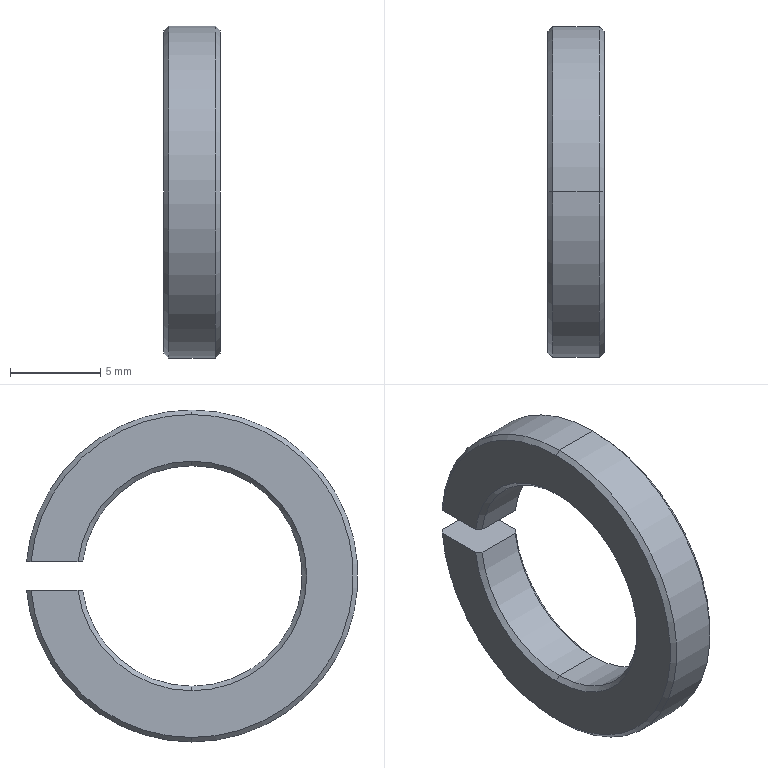Component | SolidWorks | 12_T93-1 | 1 solid | 22 faces | box 3.1 x 18.33 x 18.37 mm | volume 438 mm3 | cone 12 | cylinder 6 | plane 4 | commonest cylinder face diameters 12.2 x3 18.367 x3 | material Plain Carbon Steel
build123d program:
from build123d import *

# Parameters (mm, degrees)
EXTRUDE1_DEPTH = 3.1
CHAMFER1_SIZE  = 0.25


with BuildPart() as part:
    # Sketch1 → Extrude1 (new body)
    with BuildSketch(Plane.XY):
        with BuildLine():
            Line((-0.775, 9.151), (-0.775, 6.051))
            ThreePointArc((-0.775, 6.051), (0, -6.1), (0.775, 6.051))
            Line((0.775, 6.051), (0.775, 9.151))
            ThreePointArc((0.775, 9.151), (0, -9.183), (-0.775, 9.151))
        make_face()
    extrude(amount=EXTRUDE1_DEPTH)

    # Chamfer1
    chamfer1_edges = [part.edges().sort_by_distance(p)[0] for p in [
        (0, -6.1, 3.1),
        (0, -9.183, 3.1),
        (0, -6.1, 0),
        (0, -9.183, 0),
    ]]
    chamfer(chamfer1_edges, length=CHAMFER1_SIZE)


solid = part.part

# Placed as in the assembly
solid = solid.moved(Location((0, 0, -53.2), (0, 90, 0)))
STEP:
#1=COLOUR_RGB('',0.7922,0.8196,0.9333);
#2=FILL_AREA_STYLE_COLOUR('',#1);
#3=FILL_AREA_STYLE('',(#2));
#4=SURFACE_STYLE_FILL_AREA(#3);
#5=SURFACE_SIDE_STYLE('',(#4));
#6=SURFACE_STYLE_USAGE(.BOTH.,#5);
#7=PRESENTATION_STYLE_ASSIGNMENT((#6));
#8=CARTESIAN_POINT('',(0.009843,0.,-2.335));
#9=VERTEX_POINT('',#8);
#10=CARTESIAN_POINT('',(0.009843,0.,-1.854));
#11=VERTEX_POINT('',#10);
#12=CARTESIAN_POINT('',(0.009843,0.,-2.094));
#13=DIRECTION('',(-1.,0.,0.));
#14=DIRECTION('',(0.,0.,1.));
#15=AXIS2_PLACEMENT_3D('',#12,#13,#14);
#16=CIRCLE('',#15,0.2402);
#17=EDGE_CURVE('',#9,#11,#16,.T.);
#18=ORIENTED_EDGE('',*,*,#17,.F.);
#19=CARTESIAN_POINT('',(0.,0.,-2.344));
#20=VERTEX_POINT('',#19);
#21=CARTESIAN_POINT('',(0.,0.,-2.344));
#22=DIRECTION('',(-0.7071,0.,-0.7071));
#23=VECTOR('',#22,39.37);
#24=LINE('',#21,#23);
#25=EDGE_CURVE('',#9,#20,#24,.T.);
#26=ORIENTED_EDGE('',*,*,#25,.T.);
#27=CARTESIAN_POINT('',(0.,0.,-1.844));
#28=VERTEX_POINT('',#27);
#29=CARTESIAN_POINT('',(0.,0.,-2.094));
#30=DIRECTION('',(1.,0.,0.));
#31=DIRECTION('',(0.,0.,1.));
#32=AXIS2_PLACEMENT_3D('',#29,#30,#31);
#33=CIRCLE('',#32,0.25);
#34=EDGE_CURVE('',#28,#20,#33,.T.);
#35=ORIENTED_EDGE('',*,*,#34,.F.);
#36=CARTESIAN_POINT('',(0.,0.,-1.844));
#37=DIRECTION('',(-0.7071,0.,0.7071));
#38=VECTOR('',#37,39.37);
#39=LINE('',#36,#38);
#40=EDGE_CURVE('',#11,#28,#39,.T.);
#41=ORIENTED_EDGE('',*,*,#40,.F.);
#42=EDGE_LOOP('',(#18,#26,#35,#41));
#43=FACE_OUTER_BOUND('',#42,.T.);
#44=CARTESIAN_POINT('',(0.,0.,-2.094));
#45=DIRECTION('',(-1.,0.,0.));
#46=DIRECTION('',(0.,0.,1.));
#47=AXIS2_PLACEMENT_3D('',#44,#45,#46);
#48=CONICAL_SURFACE('',#47,0.25,0.7854);
#49=ADVANCED_FACE('',(#43),#48,.F.);
#50=CARTESIAN_POINT('',(0.009843,0.2382,-2.064));
#51=VERTEX_POINT('',#50);
#52=CARTESIAN_POINT('',(0.009843,0.,-2.094));
#53=DIRECTION('',(-1.,0.,0.));
#54=DIRECTION('',(0.,0.,1.));
#55=AXIS2_PLACEMENT_3D('',#52,#53,#54);
#56=CIRCLE('',#55,0.2402);
#57=EDGE_CURVE('',#11,#51,#56,.T.);
#58=ORIENTED_EDGE('',*,*,#57,.F.);
#59=ORIENTED_EDGE('',*,*,#40,.T.);
#60=CARTESIAN_POINT('',(0.,0.2481,-2.064));
#61=VERTEX_POINT('',#60);
#62=CARTESIAN_POINT('',(0.,0.,-2.094));
#63=DIRECTION('',(1.,0.,0.));
#64=DIRECTION('',(0.,0.,1.));
#65=AXIS2_PLACEMENT_3D('',#62,#63,#64);
#66=CIRCLE('',#65,0.25);
#67=EDGE_CURVE('',#61,#28,#66,.T.);
#68=ORIENTED_EDGE('',*,*,#67,.F.);
#69=CARTESIAN_POINT('',(0.009843,0.2382,-2.064));
#70=CARTESIAN_POINT('',(0.006562,0.2415,-2.064));
#71=CARTESIAN_POINT('',(0.003281,0.2448,-2.064));
#72=CARTESIAN_POINT('',(0.,0.2481,-2.064));
#73=B_SPLINE_CURVE_WITH_KNOTS('',3,(#69,#70,#71,#72),.UNSPECIFIED.,.F.,.F.,(4,4),(0.,0.0003549),.UNSPECIFIED.);
#74=EDGE_CURVE('',#51,#61,#73,.T.);
#75=ORIENTED_EDGE('',*,*,#74,.F.);
#76=EDGE_LOOP('',(#58,#59,#68,#75));
#77=FACE_OUTER_BOUND('',#76,.T.);
#78=CARTESIAN_POINT('',(0.,0.,-2.094));
#79=DIRECTION('',(-1.,0.,0.));
#80=DIRECTION('',(0.,0.,1.));
#81=AXIS2_PLACEMENT_3D('',#78,#79,#80);
#82=CONICAL_SURFACE('',#81,0.25,0.7854);
#83=ADVANCED_FACE('',(#77),#82,.F.);
#84=CARTESIAN_POINT('',(0.1122,0.,-1.854));
#85=VERTEX_POINT('',#84);
#86=CARTESIAN_POINT('',(0.1122,0.,-2.335));
#87=VERTEX_POINT('',#86);
#88=CARTESIAN_POINT('',(0.1122,0.,-2.094));
#89=DIRECTION('',(1.,0.,0.));
#90=DIRECTION('',(0.,0.,1.));
#91=AXIS2_PLACEMENT_3D('',#88,#89,#90);
#92=CIRCLE('',#91,0.2402);
#93=EDGE_CURVE('',#85,#87,#92,.T.);
#94=ORIENTED_EDGE('',*,*,#93,.F.);
#95=CARTESIAN_POINT('',(0.122,0.,-1.844));
#96=VERTEX_POINT('',#95);
#97=CARTESIAN_POINT('',(0.1122,0.,-1.854));
#98=DIRECTION('',(0.7071,0.,0.7071));
#99=VECTOR('',#98,39.37);
#100=LINE('',#97,#99);
#101=EDGE_CURVE('',#85,#96,#100,.T.);
#102=ORIENTED_EDGE('',*,*,#101,.T.);
#103=CARTESIAN_POINT('',(0.122,0.,-2.344));
#104=VERTEX_POINT('',#103);
#105=CARTESIAN_POINT('',(0.122,0.,-2.094));
#106=DIRECTION('',(-1.,0.,0.));
#107=DIRECTION('',(0.,0.,1.));
#108=AXIS2_PLACEMENT_3D('',#105,#106,#107);
#109=CIRCLE('',#108,0.25);
#110=EDGE_CURVE('',#104,#96,#109,.T.);
#111=ORIENTED_EDGE('',*,*,#110,.F.);
#112=CARTESIAN_POINT('',(0.1122,0.,-2.335));
#113=DIRECTION('',(0.7071,0.,-0.7071));
#114=VECTOR('',#113,39.37);
#115=LINE('',#112,#114);
#116=EDGE_CURVE('',#87,#104,#115,.T.);
#117=ORIENTED_EDGE('',*,*,#116,.F.);
#118=EDGE_LOOP('',(#94,#102,#111,#117));
#119=FACE_OUTER_BOUND('',#118,.T.);
#120=CARTESIAN_POINT('',(0.1122,0.,-2.094));
#121=DIRECTION('',(1.,0.,0.));
#122=DIRECTION('',(0.,0.,-1.));
#123=AXIS2_PLACEMENT_3D('',#120,#121,#122);
#124=CONICAL_SURFACE('',#123,0.2402,0.7854);
#125=ADVANCED_FACE('',(#119),#124,.F.);
#126=CARTESIAN_POINT('',(0.1122,0.2382,-2.125));
#127=VERTEX_POINT('',#126);
#128=CARTESIAN_POINT('',(0.1122,0.,-2.094));
#129=DIRECTION('',(1.,0.,0.));
#130=DIRECTION('',(0.,0.,1.));
#131=AXIS2_PLACEMENT_3D('',#128,#129,#130);
#132=CIRCLE('',#131,0.2402);
#133=EDGE_CURVE('',#87,#127,#132,.T.);
#134=ORIENTED_EDGE('',*,*,#133,.F.);
#135=ORIENTED_EDGE('',*,*,#116,.T.);
#136=CARTESIAN_POINT('',(0.122,0.2481,-2.125));
#137=VERTEX_POINT('',#136);
#138=CARTESIAN_POINT('',(0.122,0.,-2.094));
#139=DIRECTION('',(-1.,0.,0.));
#140=DIRECTION('',(0.,0.,1.));
#141=AXIS2_PLACEMENT_3D('',#138,#139,#140);
#142=CIRCLE('',#141,0.25);
#143=EDGE_CURVE('',#137,#104,#142,.T.);
#144=ORIENTED_EDGE('',*,*,#143,.F.);
#145=CARTESIAN_POINT('',(0.1122,0.2382,-2.125));
#146=CARTESIAN_POINT('',(0.1155,0.2415,-2.125));
#147=CARTESIAN_POINT('',(0.1188,0.2448,-2.125));
#148=CARTESIAN_POINT('',(0.122,0.2481,-2.125));
#149=B_SPLINE_CURVE_WITH_KNOTS('',3,(#145,#146,#147,#148),.UNSPECIFIED.,.F.,.F.,(4,4),(0.,0.0003549),.UNSPECIFIED.);
#150=EDGE_CURVE('',#127,#137,#149,.T.);
#151=ORIENTED_EDGE('',*,*,#150,.F.);
#152=EDGE_LOOP('',(#134,#135,#144,#151));
#153=FACE_OUTER_BOUND('',#152,.T.);
#154=CARTESIAN_POINT('',(0.1122,0.,-2.094));
#155=DIRECTION('',(1.,0.,0.));
#156=DIRECTION('',(0.,0.,-1.));
#157=AXIS2_PLACEMENT_3D('',#154,#155,#156);
#158=CONICAL_SURFACE('',#157,0.2402,0.7854);
#159=ADVANCED_FACE('',(#153),#158,.F.);
#160=CARTESIAN_POINT('',(0.,0.,-1.743));
#161=VERTEX_POINT('',#160);
#162=CARTESIAN_POINT('',(0.,0.3504,-2.064));
#163=VERTEX_POINT('',#162);
#164=CARTESIAN_POINT('',(0.,0.,-2.094));
#165=DIRECTION('',(-1.,0.,0.));
#166=DIRECTION('',(0.,0.,1.));
#167=AXIS2_PLACEMENT_3D('',#164,#165,#166);
#168=CIRCLE('',#167,0.3517);
#169=EDGE_CURVE('',#161,#163,#168,.T.);
#170=ORIENTED_EDGE('',*,*,#169,.F.);
#171=CARTESIAN_POINT('',(0.009843,0.,-1.733));
#172=VERTEX_POINT('',#171);
#173=CARTESIAN_POINT('',(0.,0.,-1.743));
#174=DIRECTION('',(0.7071,0.,0.7071));
#175=VECTOR('',#174,39.37);
#176=LINE('',#173,#175);
#177=EDGE_CURVE('',#161,#172,#176,.T.);
#178=ORIENTED_EDGE('',*,*,#177,.T.);
#179=CARTESIAN_POINT('',(0.009843,0.3603,-2.064));
#180=VERTEX_POINT('',#179);
#181=CARTESIAN_POINT('',(0.009843,0.,-2.094));
#182=DIRECTION('',(1.,0.,0.));
#183=DIRECTION('',(0.,-0.,1.));
#184=AXIS2_PLACEMENT_3D('',#181,#182,#183);
#185=CIRCLE('',#184,0.3615);
#186=EDGE_CURVE('',#180,#172,#185,.T.);
#187=ORIENTED_EDGE('',*,*,#186,.F.);
#188=CARTESIAN_POINT('',(0.,0.3504,-2.064));
#189=CARTESIAN_POINT('',(0.003281,0.3537,-2.064));
#190=CARTESIAN_POINT('',(0.006562,0.357,-2.064));
#191=CARTESIAN_POINT('',(0.009843,0.3603,-2.064));
#192=B_SPLINE_CURVE_WITH_KNOTS('',3,(#188,#189,#190,#191),.UNSPECIFIED.,.F.,.F.,(4,4),(0.,0.0003542),.UNSPECIFIED.);
#193=EDGE_CURVE('',#163,#180,#192,.T.);
#194=ORIENTED_EDGE('',*,*,#193,.F.);
#195=EDGE_LOOP('',(#170,#178,#187,#194));
#196=FACE_OUTER_BOUND('',#195,.T.);
#197=CARTESIAN_POINT('',(0.,0.,-2.094));
#198=DIRECTION('',(1.,0.,0.));
#199=DIRECTION('',(0.,0.,-1.));
#200=AXIS2_PLACEMENT_3D('',#197,#198,#199);
#201=CONICAL_SURFACE('',#200,0.3517,0.7854);
#202=ADVANCED_FACE('',(#196),#201,.T.);
#203=ORIENTED_EDGE('',*,*,#177,.F.);
#204=CARTESIAN_POINT('',(0.,0.,-2.446));
#205=VERTEX_POINT('',#204);
#206=CARTESIAN_POINT('',(0.,0.,-2.094));
#207=DIRECTION('',(-1.,0.,0.));
#208=DIRECTION('',(0.,0.,1.));
#209=AXIS2_PLACEMENT_3D('',#206,#207,#208);
#210=CIRCLE('',#209,0.3517);
#211=EDGE_CURVE('',#205,#161,#210,.T.);
#212=ORIENTED_EDGE('',*,*,#211,.F.);
#213=CARTESIAN_POINT('',(0.009843,0.,-2.456));
#214=VERTEX_POINT('',#213);
#215=CARTESIAN_POINT('',(0.,0.,-2.446));
#216=DIRECTION('',(0.7071,0.,-0.7071));
#217=VECTOR('',#216,39.37);
#218=LINE('',#215,#217);
#219=EDGE_CURVE('',#205,#214,#218,.T.);
#220=ORIENTED_EDGE('',*,*,#219,.T.);
#221=CARTESIAN_POINT('',(0.009843,0.,-2.094));
#222=DIRECTION('',(1.,0.,0.));
#223=DIRECTION('',(0.,0.,1.));
#224=AXIS2_PLACEMENT_3D('',#221,#222,#223);
#225=CIRCLE('',#224,0.3615);
#226=EDGE_CURVE('',#172,#214,#225,.T.);
#227=ORIENTED_EDGE('',*,*,#226,.F.);
#228=EDGE_LOOP('',(#203,#212,#220,#227));
#229=FACE_OUTER_BOUND('',#228,.T.);
#230=CARTESIAN_POINT('',(0.,0.,-2.094));
#231=DIRECTION('',(1.,0.,0.));
#232=DIRECTION('',(0.,0.,-1.));
#233=AXIS2_PLACEMENT_3D('',#230,#231,#232);
#234=CONICAL_SURFACE('',#233,0.3517,0.7854);
#235=ADVANCED_FACE('',(#229),#234,.T.);
#236=CARTESIAN_POINT('',(0.122,0.,-2.446));
#237=VERTEX_POINT('',#236);
#238=CARTESIAN_POINT('',(0.122,0.3504,-2.125));
#239=VERTEX_POINT('',#238);
#240=CARTESIAN_POINT('',(0.122,0.,-2.094));
#241=DIRECTION('',(1.,0.,0.));
#242=DIRECTION('',(0.,0.,1.));
#243=AXIS2_PLACEMENT_3D('',#240,#241,#242);
#244=CIRCLE('',#243,0.3517);
#245=EDGE_CURVE('',#237,#239,#244,.T.);
#246=ORIENTED_EDGE('',*,*,#245,.F.);
#247=CARTESIAN_POINT('',(0.1122,0.,-2.456));
#248=VERTEX_POINT('',#247);
#249=CARTESIAN_POINT('',(0.1122,0.,-2.456));
#250=DIRECTION('',(-0.7071,0.,-0.7071));
#251=VECTOR('',#250,39.37);
#252=LINE('',#249,#251);
#253=EDGE_CURVE('',#237,#248,#252,.T.);
#254=ORIENTED_EDGE('',*,*,#253,.T.);
#255=CARTESIAN_POINT('',(0.1122,0.3603,-2.125));
#256=VERTEX_POINT('',#255);
#257=CARTESIAN_POINT('',(0.1122,0.,-2.094));
#258=DIRECTION('',(-1.,0.,0.));
#259=DIRECTION('',(0.,0.,1.));
#260=AXIS2_PLACEMENT_3D('',#257,#258,#259);
#261=CIRCLE('',#260,0.3615);
#262=EDGE_CURVE('',#256,#248,#261,.T.);
#263=ORIENTED_EDGE('',*,*,#262,.F.);
#264=CARTESIAN_POINT('',(0.122,0.3504,-2.125));
#265=CARTESIAN_POINT('',(0.1188,0.3537,-2.125));
#266=CARTESIAN_POINT('',(0.1155,0.357,-2.125));
#267=CARTESIAN_POINT('',(0.1122,0.3603,-2.125));
#268=B_SPLINE_CURVE_WITH_KNOTS('',3,(#264,#265,#266,#267),.UNSPECIFIED.,.F.,.F.,(4,4),(0.,0.0003542),.UNSPECIFIED.);
#269=EDGE_CURVE('',#239,#256,#268,.T.);
#270=ORIENTED_EDGE('',*,*,#269,.F.);
#271=EDGE_LOOP('',(#246,#254,#263,#270));
#272=FACE_OUTER_BOUND('',#271,.T.);
#273=CARTESIAN_POINT('',(0.1122,0.,-2.094));
#274=DIRECTION('',(-1.,0.,0.));
#275=DIRECTION('',(0.,0.,1.));
#276=AXIS2_PLACEMENT_3D('',#273,#274,#275);
#277=CONICAL_SURFACE('',#276,0.3615,0.7854);
#278=ADVANCED_FACE('',(#272),#277,.T.);
#279=ORIENTED_EDGE('',*,*,#253,.F.);
#280=CARTESIAN_POINT('',(0.122,0.,-1.743));
#281=VERTEX_POINT('',#280);
#282=CARTESIAN_POINT('',(0.122,0.,-2.094));
#283=DIRECTION('',(1.,0.,0.));
#284=DIRECTION('',(0.,0.,1.));
#285=AXIS2_PLACEMENT_3D('',#282,#283,#284);
#286=CIRCLE('',#285,0.3517);
#287=EDGE_CURVE('',#281,#237,#286,.T.);
#288=ORIENTED_EDGE('',*,*,#287,.F.);
#289=CARTESIAN_POINT('',(0.1122,0.,-1.733));
#290=VERTEX_POINT('',#289);
#291=CARTESIAN_POINT('',(0.1122,0.,-1.733));
#292=DIRECTION('',(-0.7071,0.,0.7071));
#293=VECTOR('',#292,39.37);
#294=LINE('',#291,#293);
#295=EDGE_CURVE('',#281,#290,#294,.T.);
#296=ORIENTED_EDGE('',*,*,#295,.T.);
#297=CARTESIAN_POINT('',(0.1122,0.,-2.094));
#298=DIRECTION('',(-1.,0.,0.));
#299=DIRECTION('',(0.,0.,1.));
#300=AXIS2_PLACEMENT_3D('',#297,#298,#299);
#301=CIRCLE('',#300,0.3615);
#302=EDGE_CURVE('',#248,#290,#301,.T.);
#303=ORIENTED_EDGE('',*,*,#302,.F.);
#304=EDGE_LOOP('',(#279,#288,#296,#303));
#305=FACE_OUTER_BOUND('',#304,.T.);
#306=CARTESIAN_POINT('',(0.1122,0.,-2.094));
#307=DIRECTION('',(-1.,0.,0.));
#308=DIRECTION('',(0.,0.,1.));
#309=AXIS2_PLACEMENT_3D('',#306,#307,#308);
#310=CONICAL_SURFACE('',#309,0.3615,0.7854);
#311=ADVANCED_FACE('',(#305),#310,.T.);
#312=ORIENTED_EDGE('',*,*,#17,.T.);
#313=CARTESIAN_POINT('',(0.,0.,-1.854));
#314=DIRECTION('',(1.,0.,0.));
#315=VECTOR('',#314,39.37);
#316=LINE('',#313,#315);
#317=EDGE_CURVE('',#11,#85,#316,.T.);
#318=ORIENTED_EDGE('',*,*,#317,.T.);
#319=ORIENTED_EDGE('',*,*,#93,.T.);
#320=CARTESIAN_POINT('',(0.,0.,-2.335));
#321=DIRECTION('',(1.,0.,0.));
#322=VECTOR('',#321,39.37);
#323=LINE('',#320,#322);
#324=EDGE_CURVE('',#9,#87,#323,.T.);
#325=ORIENTED_EDGE('',*,*,#324,.F.);
#326=EDGE_LOOP('',(#312,#318,#319,#325));
#327=FACE_OUTER_BOUND('',#326,.T.);
#328=CARTESIAN_POINT('',(0.,0.,-2.094));
#329=DIRECTION('',(1.,0.,0.));
#330=DIRECTION('',(0.,0.,-1.));
#331=AXIS2_PLACEMENT_3D('',#328,#329,#330);
#332=CYLINDRICAL_SURFACE('',#331,0.2402);
#333=ADVANCED_FACE('',(#327),#332,.F.);
#334=CARTESIAN_POINT('',(0.009843,0.2382,-2.125));
#335=VERTEX_POINT('',#334);
#336=CARTESIAN_POINT('',(0.009843,0.,-2.094));
#337=DIRECTION('',(-1.,0.,0.));
#338=DIRECTION('',(0.,0.,1.));
#339=AXIS2_PLACEMENT_3D('',#336,#337,#338);
#340=CIRCLE('',#339,0.2402);
#341=EDGE_CURVE('',#335,#9,#340,.T.);
#342=ORIENTED_EDGE('',*,*,#341,.T.);
#343=ORIENTED_EDGE('',*,*,#324,.T.);
#344=ORIENTED_EDGE('',*,*,#133,.T.);
#345=CARTESIAN_POINT('',(0.,0.2382,-2.125));
#346=DIRECTION('',(1.,0.,0.));
#347=VECTOR('',#346,39.37);
#348=LINE('',#345,#347);
#349=EDGE_CURVE('',#335,#127,#348,.T.);
#350=ORIENTED_EDGE('',*,*,#349,.F.);
#351=EDGE_LOOP('',(#342,#343,#344,#350));
#352=FACE_OUTER_BOUND('',#351,.T.);
#353=CARTESIAN_POINT('',(0.,0.,-2.094));
#354=DIRECTION('',(1.,0.,0.));
#355=DIRECTION('',(0.,0.,-1.));
#356=AXIS2_PLACEMENT_3D('',#353,#354,#355);
#357=CYLINDRICAL_SURFACE('',#356,0.2402);
#358=ADVANCED_FACE('',(#352),#357,.F.);
#359=ORIENTED_EDGE('',*,*,#186,.T.);
#360=CARTESIAN_POINT('',(0.,0.,-1.733));
#361=DIRECTION('',(1.,0.,0.));
#362=VECTOR('',#361,39.37);
#363=LINE('',#360,#362);
#364=EDGE_CURVE('',#172,#290,#363,.T.);
#365=ORIENTED_EDGE('',*,*,#364,.T.);
#366=CARTESIAN_POINT('',(0.1122,0.3603,-2.064));
#367=VERTEX_POINT('',#366);
#368=CARTESIAN_POINT('',(0.1122,0.,-2.094));
#369=DIRECTION('',(-1.,0.,0.));
#370=DIRECTION('',(0.,0.,1.));
#371=AXIS2_PLACEMENT_3D('',#368,#369,#370);
#372=CIRCLE('',#371,0.3615);
#373=EDGE_CURVE('',#290,#367,#372,.T.);
#374=ORIENTED_EDGE('',*,*,#373,.T.);
#375=CARTESIAN_POINT('',(0.,0.3603,-2.064));
#376=DIRECTION('',(1.,0.,0.));
#377=VECTOR('',#376,39.37);
#378=LINE('',#375,#377);
#379=EDGE_CURVE('',#180,#367,#378,.T.);
#380=ORIENTED_EDGE('',*,*,#379,.F.);
#381=EDGE_LOOP('',(#359,#365,#374,#380));
#382=FACE_OUTER_BOUND('',#381,.T.);
#383=CARTESIAN_POINT('',(0.,0.,-2.094));
#384=DIRECTION('',(1.,0.,0.));
#385=DIRECTION('',(0.,0.,-1.));
#386=AXIS2_PLACEMENT_3D('',#383,#384,#385);
#387=CYLINDRICAL_SURFACE('',#386,0.3615);
#388=ADVANCED_FACE('',(#382),#387,.T.);
#389=ORIENTED_EDGE('',*,*,#364,.F.);
#390=ORIENTED_EDGE('',*,*,#226,.T.);
#391=CARTESIAN_POINT('',(0.,0.,-2.456));
#392=DIRECTION('',(1.,0.,0.));
#393=VECTOR('',#392,39.37);
#394=LINE('',#391,#393);
#395=EDGE_CURVE('',#214,#248,#394,.T.);
#396=ORIENTED_EDGE('',*,*,#395,.T.);
#397=ORIENTED_EDGE('',*,*,#302,.T.);
#398=EDGE_LOOP('',(#389,#390,#396,#397));
#399=FACE_OUTER_BOUND('',#398,.T.);
#400=CARTESIAN_POINT('',(0.,0.,-2.094));
#401=DIRECTION('',(1.,0.,0.));
#402=DIRECTION('',(0.,0.,-1.));
#403=AXIS2_PLACEMENT_3D('',#400,#401,#402);
#404=CYLINDRICAL_SURFACE('',#403,0.3615);
#405=ADVANCED_FACE('',(#399),#404,.T.);
#406=ORIENTED_EDGE('',*,*,#395,.F.);
#407=CARTESIAN_POINT('',(0.009843,0.3603,-2.125));
#408=VERTEX_POINT('',#407);
#409=CARTESIAN_POINT('',(0.009843,0.,-2.094));
#410=DIRECTION('',(1.,0.,0.));
#411=DIRECTION('',(0.,0.,1.));
#412=AXIS2_PLACEMENT_3D('',#409,#410,#411);
#413=CIRCLE('',#412,0.3615);
#414=EDGE_CURVE('',#214,#408,#413,.T.);
#415=ORIENTED_EDGE('',*,*,#414,.T.);
#416=CARTESIAN_POINT('',(0.,0.3603,-2.125));
#417=DIRECTION('',(1.,0.,0.));
#418=VECTOR('',#417,39.37);
#419=LINE('',#416,#418);
#420=EDGE_CURVE('',#408,#256,#419,.T.);
#421=ORIENTED_EDGE('',*,*,#420,.T.);
#422=ORIENTED_EDGE('',*,*,#262,.T.);
#423=EDGE_LOOP('',(#406,#415,#421,#422));
#424=FACE_OUTER_BOUND('',#423,.T.);
#425=CARTESIAN_POINT('',(0.,0.,-2.094));
#426=DIRECTION('',(1.,0.,0.));
#427=DIRECTION('',(0.,0.,-1.));
#428=AXIS2_PLACEMENT_3D('',#425,#426,#427);
#429=CYLINDRICAL_SURFACE('',#428,0.3615);
#430=ADVANCED_FACE('',(#424),#429,.T.);
#431=ORIENTED_EDGE('',*,*,#379,.T.);
#432=CARTESIAN_POINT('',(0.122,0.3504,-2.064));
#433=VERTEX_POINT('',#432);
#434=CARTESIAN_POINT('',(0.1122,0.3603,-2.064));
#435=CARTESIAN_POINT('',(0.1155,0.357,-2.064));
#436=CARTESIAN_POINT('',(0.1188,0.3537,-2.064));
#437=CARTESIAN_POINT('',(0.122,0.3504,-2.064));
#438=B_SPLINE_CURVE_WITH_KNOTS('',3,(#434,#435,#436,#437),.UNSPECIFIED.,.F.,.F.,(4,4),(0.,0.0003542),.UNSPECIFIED.);
#439=EDGE_CURVE('',#367,#433,#438,.T.);
#440=ORIENTED_EDGE('',*,*,#439,.T.);
#441=CARTESIAN_POINT('',(0.122,0.2481,-2.064));
#442=VERTEX_POINT('',#441);
#443=CARTESIAN_POINT('',(0.122,0.3603,-2.064));
#444=DIRECTION('',(0.,-1.,0.));
#445=VECTOR('',#444,39.37);
#446=LINE('',#443,#445);
#447=EDGE_CURVE('',#433,#442,#446,.T.);
#448=ORIENTED_EDGE('',*,*,#447,.T.);
#449=CARTESIAN_POINT('',(0.1122,0.2382,-2.064));
#450=VERTEX_POINT('',#449);
#451=CARTESIAN_POINT('',(0.122,0.2481,-2.064));
#452=CARTESIAN_POINT('',(0.1188,0.2448,-2.064));
#453=CARTESIAN_POINT('',(0.1155,0.2415,-2.064));
#454=CARTESIAN_POINT('',(0.1122,0.2382,-2.064));
#455=B_SPLINE_CURVE_WITH_KNOTS('',3,(#451,#452,#453,#454),.UNSPECIFIED.,.F.,.F.,(4,4),(0.,0.0003549),.UNSPECIFIED.);
#456=EDGE_CURVE('',#442,#450,#455,.T.);
#457=ORIENTED_EDGE('',*,*,#456,.T.);
#458=CARTESIAN_POINT('',(0.,0.2382,-2.064));
#459=DIRECTION('',(1.,0.,0.));
#460=VECTOR('',#459,39.37);
#461=LINE('',#458,#460);
#462=EDGE_CURVE('',#51,#450,#461,.T.);
#463=ORIENTED_EDGE('',*,*,#462,.F.);
#464=ORIENTED_EDGE('',*,*,#74,.T.);
#465=CARTESIAN_POINT('',(0.,0.3603,-2.064));
#466=DIRECTION('',(0.,-1.,0.));
#467=VECTOR('',#466,39.37);
#468=LINE('',#465,#467);
#469=EDGE_CURVE('',#163,#61,#468,.T.);
#470=ORIENTED_EDGE('',*,*,#469,.F.);
#471=ORIENTED_EDGE('',*,*,#193,.T.);
#472=EDGE_LOOP('',(#431,#440,#448,#457,#463,#464,#470,#471));
#473=FACE_OUTER_BOUND('',#472,.T.);
#474=CARTESIAN_POINT('',(0.,0.3603,-2.064));
#475=DIRECTION('',(0.,0.,1.));
#476=DIRECTION('',(1.,0.,0.));
#477=AXIS2_PLACEMENT_3D('',#474,#475,#476);
#478=PLANE('',#477);
#479=ADVANCED_FACE('',(#473),#478,.F.);
#480=ORIENTED_EDGE('',*,*,#317,.F.);
#481=ORIENTED_EDGE('',*,*,#57,.T.);
#482=ORIENTED_EDGE('',*,*,#462,.T.);
#483=CARTESIAN_POINT('',(0.1122,0.,-2.094));
#484=DIRECTION('',(1.,0.,0.));
#485=DIRECTION('',(0.,-0.,1.));
#486=AXIS2_PLACEMENT_3D('',#483,#484,#485);
#487=CIRCLE('',#486,0.2402);
#488=EDGE_CURVE('',#450,#85,#487,.T.);
#489=ORIENTED_EDGE('',*,*,#488,.T.);
#490=EDGE_LOOP('',(#480,#481,#482,#489));
#491=FACE_OUTER_BOUND('',#490,.T.);
#492=CARTESIAN_POINT('',(0.,0.,-2.094));
#493=DIRECTION('',(1.,0.,0.));
#494=DIRECTION('',(0.,0.,-1.));
#495=AXIS2_PLACEMENT_3D('',#492,#493,#494);
#496=CYLINDRICAL_SURFACE('',#495,0.2402);
#497=ADVANCED_FACE('',(#491),#496,.F.);
#498=CARTESIAN_POINT('',(0.122,0.3603,-2.125));
#499=DIRECTION('',(0.,1.,0.));
#500=VECTOR('',#499,39.37);
#501=LINE('',#498,#500);
#502=EDGE_CURVE('',#137,#239,#501,.T.);
#503=ORIENTED_EDGE('',*,*,#502,.T.);
#504=ORIENTED_EDGE('',*,*,#269,.T.);
#505=ORIENTED_EDGE('',*,*,#420,.F.);
#506=CARTESIAN_POINT('',(0.,0.3504,-2.125));
#507=VERTEX_POINT('',#506);
#508=CARTESIAN_POINT('',(0.009843,0.3603,-2.125));
#509=CARTESIAN_POINT('',(0.006562,0.357,-2.125));
#510=CARTESIAN_POINT('',(0.003281,0.3537,-2.125));
#511=CARTESIAN_POINT('',(0.,0.3504,-2.125));
#512=B_SPLINE_CURVE_WITH_KNOTS('',3,(#508,#509,#510,#511),.UNSPECIFIED.,.F.,.F.,(4,4),(0.,0.0003542),.UNSPECIFIED.);
#513=EDGE_CURVE('',#408,#507,#512,.T.);
#514=ORIENTED_EDGE('',*,*,#513,.T.);
#515=CARTESIAN_POINT('',(0.,0.2481,-2.125));
#516=VERTEX_POINT('',#515);
#517=CARTESIAN_POINT('',(0.,0.3603,-2.125));
#518=DIRECTION('',(0.,1.,0.));
#519=VECTOR('',#518,39.37);
#520=LINE('',#517,#519);
#521=EDGE_CURVE('',#516,#507,#520,.T.);
#522=ORIENTED_EDGE('',*,*,#521,.F.);
#523=CARTESIAN_POINT('',(0.,0.2481,-2.125));
#524=CARTESIAN_POINT('',(0.003281,0.2448,-2.125));
#525=CARTESIAN_POINT('',(0.006562,0.2415,-2.125));
#526=CARTESIAN_POINT('',(0.009843,0.2382,-2.125));
#527=B_SPLINE_CURVE_WITH_KNOTS('',3,(#523,#524,#525,#526),.UNSPECIFIED.,.F.,.F.,(4,4),(0.,0.0003549),.UNSPECIFIED.);
#528=EDGE_CURVE('',#516,#335,#527,.T.);
#529=ORIENTED_EDGE('',*,*,#528,.T.);
#530=ORIENTED_EDGE('',*,*,#349,.T.);
#531=ORIENTED_EDGE('',*,*,#150,.T.);
#532=EDGE_LOOP('',(#503,#504,#505,#514,#522,#529,#530,#531));
#533=FACE_OUTER_BOUND('',#532,.T.);
#534=CARTESIAN_POINT('',(0.,0.3603,-2.125));
#535=DIRECTION('',(0.,0.,-1.));
#536=DIRECTION('',(-1.,0.,0.));
#537=AXIS2_PLACEMENT_3D('',#534,#535,#536);
#538=PLANE('',#537);
#539=ADVANCED_FACE('',(#533),#538,.F.);
#540=ORIENTED_EDGE('',*,*,#521,.T.);
#541=CARTESIAN_POINT('',(0.,0.,-2.094));
#542=DIRECTION('',(-1.,0.,0.));
#543=DIRECTION('',(0.,0.,1.));
#544=AXIS2_PLACEMENT_3D('',#541,#542,#543);
#545=CIRCLE('',#544,0.3517);
#546=EDGE_CURVE('',#507,#205,#545,.T.);
#547=ORIENTED_EDGE('',*,*,#546,.T.);
#548=ORIENTED_EDGE('',*,*,#211,.T.);
#549=ORIENTED_EDGE('',*,*,#169,.T.);
#550=ORIENTED_EDGE('',*,*,#469,.T.);
#551=ORIENTED_EDGE('',*,*,#67,.T.);
#552=ORIENTED_EDGE('',*,*,#34,.T.);
#553=CARTESIAN_POINT('',(0.,0.,-2.094));
#554=DIRECTION('',(1.,0.,0.));
#555=DIRECTION('',(0.,-0.,1.));
#556=AXIS2_PLACEMENT_3D('',#553,#554,#555);
#557=CIRCLE('',#556,0.25);
#558=EDGE_CURVE('',#20,#516,#557,.T.);
#559=ORIENTED_EDGE('',*,*,#558,.T.);
#560=EDGE_LOOP('',(#540,#547,#548,#549,#550,#551,#552,#559));
#561=FACE_OUTER_BOUND('',#560,.T.);
#562=CARTESIAN_POINT('',(0.,0.,-2.094));
#563=DIRECTION('',(-1.,0.,0.));
#564=DIRECTION('',(0.,0.,1.));
#565=AXIS2_PLACEMENT_3D('',#562,#563,#564);
#566=PLANE('',#565);
#567=ADVANCED_FACE('',(#561),#566,.T.);
#568=ORIENTED_EDGE('',*,*,#447,.F.);
#569=CARTESIAN_POINT('',(0.122,0.,-2.094));
#570=DIRECTION('',(1.,0.,0.));
#571=DIRECTION('',(0.,-0.,1.));
#572=AXIS2_PLACEMENT_3D('',#569,#570,#571);
#573=CIRCLE('',#572,0.3517);
#574=EDGE_CURVE('',#433,#281,#573,.T.);
#575=ORIENTED_EDGE('',*,*,#574,.T.);
#576=ORIENTED_EDGE('',*,*,#287,.T.);
#577=ORIENTED_EDGE('',*,*,#245,.T.);
#578=ORIENTED_EDGE('',*,*,#502,.F.);
#579=ORIENTED_EDGE('',*,*,#143,.T.);
#580=ORIENTED_EDGE('',*,*,#110,.T.);
#581=CARTESIAN_POINT('',(0.122,0.,-2.094));
#582=DIRECTION('',(-1.,0.,0.));
#583=DIRECTION('',(0.,0.,1.));
#584=AXIS2_PLACEMENT_3D('',#581,#582,#583);
#585=CIRCLE('',#584,0.25);
#586=EDGE_CURVE('',#96,#442,#585,.T.);
#587=ORIENTED_EDGE('',*,*,#586,.T.);
#588=EDGE_LOOP('',(#568,#575,#576,#577,#578,#579,#580,#587));
#589=FACE_OUTER_BOUND('',#588,.T.);
#590=CARTESIAN_POINT('',(0.122,0.,-2.094));
#591=DIRECTION('',(-1.,0.,0.));
#592=DIRECTION('',(0.,0.,1.));
#593=AXIS2_PLACEMENT_3D('',#590,#591,#592);
#594=PLANE('',#593);
#595=ADVANCED_FACE('',(#589),#594,.F.);
#596=ORIENTED_EDGE('',*,*,#295,.F.);
#597=ORIENTED_EDGE('',*,*,#574,.F.);
#598=ORIENTED_EDGE('',*,*,#439,.F.);
#599=ORIENTED_EDGE('',*,*,#373,.F.);
#600=EDGE_LOOP('',(#596,#597,#598,#599));
#601=FACE_OUTER_BOUND('',#600,.T.);
#602=CARTESIAN_POINT('',(0.1122,0.,-2.094));
#603=DIRECTION('',(-1.,0.,0.));
#604=DIRECTION('',(0.,0.,1.));
#605=AXIS2_PLACEMENT_3D('',#602,#603,#604);
#606=CONICAL_SURFACE('',#605,0.3615,0.7854);
#607=ADVANCED_FACE('',(#601),#606,.T.);
#608=ORIENTED_EDGE('',*,*,#219,.F.);
#609=ORIENTED_EDGE('',*,*,#546,.F.);
#610=ORIENTED_EDGE('',*,*,#513,.F.);
#611=ORIENTED_EDGE('',*,*,#414,.F.);
#612=EDGE_LOOP('',(#608,#609,#610,#611));
#613=FACE_OUTER_BOUND('',#612,.T.);
#614=CARTESIAN_POINT('',(0.,0.,-2.094));
#615=DIRECTION('',(1.,0.,0.));
#616=DIRECTION('',(0.,0.,-1.));
#617=AXIS2_PLACEMENT_3D('',#614,#615,#616);
#618=CONICAL_SURFACE('',#617,0.3517,0.7854);
#619=ADVANCED_FACE('',(#613),#618,.T.);
#620=ORIENTED_EDGE('',*,*,#101,.F.);
#621=ORIENTED_EDGE('',*,*,#488,.F.);
#622=ORIENTED_EDGE('',*,*,#456,.F.);
#623=ORIENTED_EDGE('',*,*,#586,.F.);
#624=EDGE_LOOP('',(#620,#621,#622,#623));
#625=FACE_OUTER_BOUND('',#624,.T.);
#626=CARTESIAN_POINT('',(0.1122,0.,-2.094));
#627=DIRECTION('',(1.,0.,0.));
#628=DIRECTION('',(0.,0.,-1.));
#629=AXIS2_PLACEMENT_3D('',#626,#627,#628);
#630=CONICAL_SURFACE('',#629,0.2402,0.7854);
#631=ADVANCED_FACE('',(#625),#630,.F.);
#632=ORIENTED_EDGE('',*,*,#25,.F.);
#633=ORIENTED_EDGE('',*,*,#341,.F.);
#634=ORIENTED_EDGE('',*,*,#528,.F.);
#635=ORIENTED_EDGE('',*,*,#558,.F.);
#636=EDGE_LOOP('',(#632,#633,#634,#635));
#637=FACE_OUTER_BOUND('',#636,.T.);
#638=CARTESIAN_POINT('',(0.,0.,-2.094));
#639=DIRECTION('',(-1.,0.,0.));
#640=DIRECTION('',(0.,0.,1.));
#641=AXIS2_PLACEMENT_3D('',#638,#639,#640);
#642=CONICAL_SURFACE('',#641,0.25,0.7854);
#643=ADVANCED_FACE('',(#637),#642,.F.);
#644=CLOSED_SHELL('',(#49,#83,#125,#159,#202,#235,#278,#311,#333,#358,#388,#405,#430,#479,#497,#539,#567,#595,#607,#619,#631,#643));
#645=MANIFOLD_SOLID_BREP('',#644);
#646=STYLED_ITEM('',(#7),#645);
#647=(LENGTH_UNIT()NAMED_UNIT(*)SI_UNIT($,.METRE.));
#648=LENGTH_MEASURE_WITH_UNIT(LENGTH_MEASURE(0.0254),#647);
#649=DIMENSIONAL_EXPONENTS(1.,0.,0.,0.,0.,0.,0.);
#650=(CONVERSION_BASED_UNIT('',#648)LENGTH_UNIT()NAMED_UNIT(#649));
#651=UNCERTAINTY_MEASURE_WITH_UNIT(LENGTH_MEASURE(0.00001),#650,'','');
#652=(NAMED_UNIT(*)PLANE_ANGLE_UNIT()SI_UNIT($,.RADIAN.));
#653=(NAMED_UNIT(*)SI_UNIT($,.STERADIAN.)SOLID_ANGLE_UNIT());
#654=(GEOMETRIC_REPRESENTATION_CONTEXT(3)GLOBAL_UNCERTAINTY_ASSIGNED_CONTEXT((#651))GLOBAL_UNIT_ASSIGNED_CONTEXT((#650,#652,#653))REPRESENTATION_CONTEXT('',''));
#655=MECHANICAL_DESIGN_GEOMETRIC_PRESENTATION_REPRESENTATION('',(#646),#654);
#656=PRESENTATION_LAYER_ASSIGNMENT('','',(#646));
#657=CARTESIAN_POINT('',(0.,0.,0.));
#658=DIRECTION('',(0.,0.,1.));
#659=DIRECTION('',(1.,0.,0.));
#660=AXIS2_PLACEMENT_3D('',#657,#658,#659);
#661=(LENGTH_UNIT()NAMED_UNIT(*)SI_UNIT($,.METRE.));
#662=LENGTH_MEASURE_WITH_UNIT(LENGTH_MEASURE(0.0254),#661);
#663=DIMENSIONAL_EXPONENTS(1.,0.,0.,0.,0.,0.,0.);
#664=(CONVERSION_BASED_UNIT('',#662)LENGTH_UNIT()NAMED_UNIT(#663));
#665=UNCERTAINTY_MEASURE_WITH_UNIT(LENGTH_MEASURE(0.00001),#664,'','');
#666=(NAMED_UNIT(*)PLANE_ANGLE_UNIT()SI_UNIT($,.RADIAN.));
#667=(NAMED_UNIT(*)SI_UNIT($,.STERADIAN.)SOLID_ANGLE_UNIT());
#668=(GEOMETRIC_REPRESENTATION_CONTEXT(3)GLOBAL_UNCERTAINTY_ASSIGNED_CONTEXT((#665))GLOBAL_UNIT_ASSIGNED_CONTEXT((#664,#666,#667))REPRESENTATION_CONTEXT('',''));
#669=ADVANCED_BREP_SHAPE_REPRESENTATION('',(#645,#660),#668);